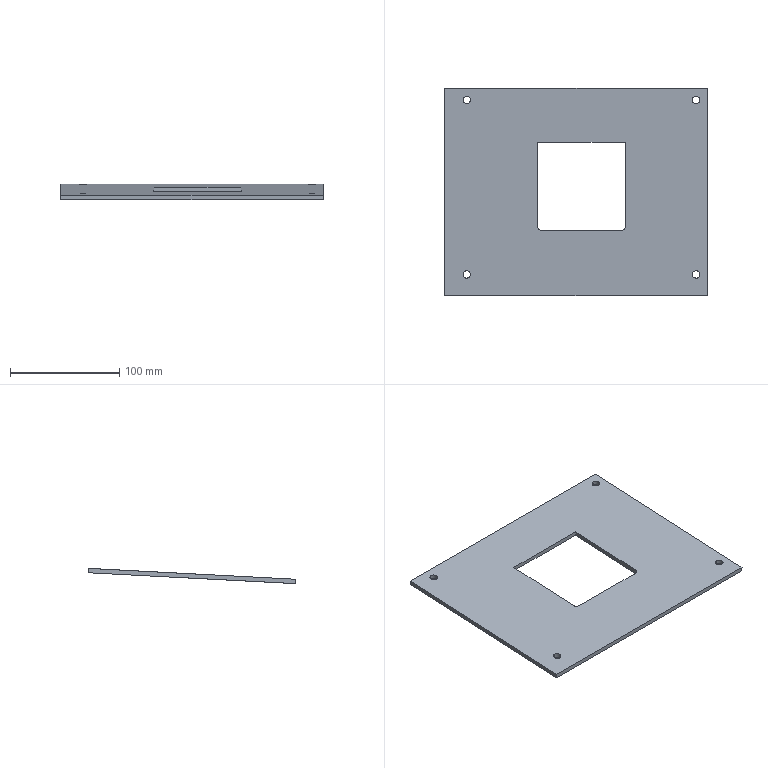Component | SolidWorks | YC1-315HangingBoxOverall-1_YC1-315SupportFrameT()-1_YC1-160OperationStationBaffleT-1 | 1 solid | 20 faces | box 240 x 189.95 x 13.94 mm | volume 155860 mm3 | cylinder 10 | plane 10 | commonest cylinder face diameters 7 x8 8 x2 | material Plain Carbon Steel
STEP:
#1=COLOUR_RGB('',0.7922,0.8196,0.9333);
#2=FILL_AREA_STYLE_COLOUR('',#1);
#3=FILL_AREA_STYLE('',(#2));
#4=SURFACE_STYLE_FILL_AREA(#3);
#5=SURFACE_SIDE_STYLE('',(#4));
#6=SURFACE_STYLE_USAGE(.BOTH.,#5);
#7=PRESENTATION_STYLE_ASSIGNMENT((#6));
#8=CARTESIAN_POINT('',(33.071,65.604,2.308));
#9=VERTEX_POINT('',#8);
#10=CARTESIAN_POINT('',(33.071,65.328,2.294));
#11=VERTEX_POINT('',#10);
#12=CARTESIAN_POINT('',(33.071,65.466,2.301));
#13=DIRECTION('',(-0.,-0.05234,0.9986));
#14=DIRECTION('',(0.,-0.9986,-0.05234));
#15=AXIS2_PLACEMENT_3D('',#12,#13,#14);
#16=CIRCLE('',#15,0.1378);
#17=EDGE_CURVE('',#9,#11,#16,.T.);
#18=ORIENTED_EDGE('',*,*,#17,.F.);
#19=CARTESIAN_POINT('',(33.071,65.595,2.465));
#20=VERTEX_POINT('',#19);
#21=CARTESIAN_POINT('',(33.071,65.604,2.308));
#22=DIRECTION('',(-0.,-0.05234,0.9986));
#23=VECTOR('',#22,39.37);
#24=LINE('',#21,#23);
#25=EDGE_CURVE('',#9,#20,#24,.T.);
#26=ORIENTED_EDGE('',*,*,#25,.T.);
#27=CARTESIAN_POINT('',(33.071,65.32,2.451));
#28=VERTEX_POINT('',#27);
#29=CARTESIAN_POINT('',(33.071,65.458,2.458));
#30=DIRECTION('',(-0.,-0.05234,0.9986));
#31=DIRECTION('',(0.,-0.9986,-0.05234));
#32=AXIS2_PLACEMENT_3D('',#29,#30,#31);
#33=CIRCLE('',#32,0.1378);
#34=EDGE_CURVE('',#20,#28,#33,.T.);
#35=ORIENTED_EDGE('',*,*,#34,.T.);
#36=CARTESIAN_POINT('',(33.071,65.328,2.294));
#37=DIRECTION('',(-0.,-0.05234,0.9986));
#38=VECTOR('',#37,39.37);
#39=LINE('',#36,#38);
#40=EDGE_CURVE('',#11,#28,#39,.T.);
#41=ORIENTED_EDGE('',*,*,#40,.F.);
#42=EDGE_LOOP('',(#18,#26,#35,#41));
#43=FACE_OUTER_BOUND('',#42,.T.);
#44=CARTESIAN_POINT('',(33.071,65.466,2.301));
#45=DIRECTION('',(-0.,-0.05234,0.9986));
#46=DIRECTION('',(0.,-0.9986,-0.05234));
#47=AXIS2_PLACEMENT_3D('',#44,#45,#46);
#48=CYLINDRICAL_SURFACE('',#47,0.1378);
#49=ADVANCED_FACE('',(#43),#48,.F.);
#50=CARTESIAN_POINT('',(41.339,65.604,2.308));
#51=VERTEX_POINT('',#50);
#52=CARTESIAN_POINT('',(41.339,65.328,2.294));
#53=VERTEX_POINT('',#52);
#54=CARTESIAN_POINT('',(41.339,65.466,2.301));
#55=DIRECTION('',(-0.,-0.05234,0.9986));
#56=DIRECTION('',(0.,-0.9986,-0.05234));
#57=AXIS2_PLACEMENT_3D('',#54,#55,#56);
#58=CIRCLE('',#57,0.1378);
#59=EDGE_CURVE('',#51,#53,#58,.T.);
#60=ORIENTED_EDGE('',*,*,#59,.F.);
#61=CARTESIAN_POINT('',(41.339,65.595,2.465));
#62=VERTEX_POINT('',#61);
#63=CARTESIAN_POINT('',(41.339,65.604,2.308));
#64=DIRECTION('',(-0.,-0.05234,0.9986));
#65=VECTOR('',#64,39.37);
#66=LINE('',#63,#65);
#67=EDGE_CURVE('',#51,#62,#66,.T.);
#68=ORIENTED_EDGE('',*,*,#67,.T.);
#69=CARTESIAN_POINT('',(41.339,65.32,2.451));
#70=VERTEX_POINT('',#69);
#71=CARTESIAN_POINT('',(41.339,65.458,2.458));
#72=DIRECTION('',(-0.,-0.05234,0.9986));
#73=DIRECTION('',(0.,-0.9986,-0.05234));
#74=AXIS2_PLACEMENT_3D('',#71,#72,#73);
#75=CIRCLE('',#74,0.1378);
#76=EDGE_CURVE('',#62,#70,#75,.T.);
#77=ORIENTED_EDGE('',*,*,#76,.T.);
#78=CARTESIAN_POINT('',(41.339,65.328,2.294));
#79=DIRECTION('',(-0.,-0.05234,0.9986));
#80=VECTOR('',#79,39.37);
#81=LINE('',#78,#80);
#82=EDGE_CURVE('',#53,#70,#81,.T.);
#83=ORIENTED_EDGE('',*,*,#82,.F.);
#84=EDGE_LOOP('',(#60,#68,#77,#83));
#85=FACE_OUTER_BOUND('',#84,.T.);
#86=CARTESIAN_POINT('',(41.339,65.466,2.301));
#87=DIRECTION('',(-0.,-0.05234,0.9986));
#88=DIRECTION('',(0.,-0.9986,-0.05234));
#89=AXIS2_PLACEMENT_3D('',#86,#87,#88);
#90=CYLINDRICAL_SURFACE('',#89,0.1378);
#91=ADVANCED_FACE('',(#85),#90,.F.);
#92=CARTESIAN_POINT('',(41.339,59.313,1.978));
#93=VERTEX_POINT('',#92);
#94=CARTESIAN_POINT('',(41.339,59.038,1.964));
#95=VERTEX_POINT('',#94);
#96=CARTESIAN_POINT('',(41.339,59.175,1.971));
#97=DIRECTION('',(-0.,-0.05234,0.9986));
#98=DIRECTION('',(0.,-0.9986,-0.05234));
#99=AXIS2_PLACEMENT_3D('',#96,#97,#98);
#100=CIRCLE('',#99,0.1378);
#101=EDGE_CURVE('',#93,#95,#100,.T.);
#102=ORIENTED_EDGE('',*,*,#101,.F.);
#103=CARTESIAN_POINT('',(41.339,59.305,2.136));
#104=VERTEX_POINT('',#103);
#105=CARTESIAN_POINT('',(41.339,59.313,1.978));
#106=DIRECTION('',(-0.,-0.05234,0.9986));
#107=VECTOR('',#106,39.37);
#108=LINE('',#105,#107);
#109=EDGE_CURVE('',#93,#104,#108,.T.);
#110=ORIENTED_EDGE('',*,*,#109,.T.);
#111=CARTESIAN_POINT('',(41.339,59.03,2.121));
#112=VERTEX_POINT('',#111);
#113=CARTESIAN_POINT('',(41.339,59.167,2.128));
#114=DIRECTION('',(-0.,-0.05234,0.9986));
#115=DIRECTION('',(0.,-0.9986,-0.05234));
#116=AXIS2_PLACEMENT_3D('',#113,#114,#115);
#117=CIRCLE('',#116,0.1378);
#118=EDGE_CURVE('',#104,#112,#117,.T.);
#119=ORIENTED_EDGE('',*,*,#118,.T.);
#120=CARTESIAN_POINT('',(41.339,59.038,1.964));
#121=DIRECTION('',(-0.,-0.05234,0.9986));
#122=VECTOR('',#121,39.37);
#123=LINE('',#120,#122);
#124=EDGE_CURVE('',#95,#112,#123,.T.);
#125=ORIENTED_EDGE('',*,*,#124,.F.);
#126=EDGE_LOOP('',(#102,#110,#119,#125));
#127=FACE_OUTER_BOUND('',#126,.T.);
#128=CARTESIAN_POINT('',(41.339,59.175,1.971));
#129=DIRECTION('',(-0.,-0.05234,0.9986));
#130=DIRECTION('',(0.,-0.9986,-0.05234));
#131=AXIS2_PLACEMENT_3D('',#128,#129,#130);
#132=CYLINDRICAL_SURFACE('',#131,0.1378);
#133=ADVANCED_FACE('',(#127),#132,.F.);
#134=CARTESIAN_POINT('',(33.071,59.313,1.978));
#135=VERTEX_POINT('',#134);
#136=CARTESIAN_POINT('',(33.071,59.038,1.964));
#137=VERTEX_POINT('',#136);
#138=CARTESIAN_POINT('',(33.071,59.175,1.971));
#139=DIRECTION('',(-0.,-0.05234,0.9986));
#140=DIRECTION('',(0.,-0.9986,-0.05234));
#141=AXIS2_PLACEMENT_3D('',#138,#139,#140);
#142=CIRCLE('',#141,0.1378);
#143=EDGE_CURVE('',#135,#137,#142,.T.);
#144=ORIENTED_EDGE('',*,*,#143,.F.);
#145=CARTESIAN_POINT('',(33.071,59.305,2.136));
#146=VERTEX_POINT('',#145);
#147=CARTESIAN_POINT('',(33.071,59.313,1.978));
#148=DIRECTION('',(-0.,-0.05234,0.9986));
#149=VECTOR('',#148,39.37);
#150=LINE('',#147,#149);
#151=EDGE_CURVE('',#135,#146,#150,.T.);
#152=ORIENTED_EDGE('',*,*,#151,.T.);
#153=CARTESIAN_POINT('',(33.071,59.03,2.121));
#154=VERTEX_POINT('',#153);
#155=CARTESIAN_POINT('',(33.071,59.167,2.128));
#156=DIRECTION('',(-0.,-0.05234,0.9986));
#157=DIRECTION('',(0.,-0.9986,-0.05234));
#158=AXIS2_PLACEMENT_3D('',#155,#156,#157);
#159=CIRCLE('',#158,0.1378);
#160=EDGE_CURVE('',#146,#154,#159,.T.);
#161=ORIENTED_EDGE('',*,*,#160,.T.);
#162=CARTESIAN_POINT('',(33.071,59.038,1.964));
#163=DIRECTION('',(-0.,-0.05234,0.9986));
#164=VECTOR('',#163,39.37);
#165=LINE('',#162,#164);
#166=EDGE_CURVE('',#137,#154,#165,.T.);
#167=ORIENTED_EDGE('',*,*,#166,.F.);
#168=EDGE_LOOP('',(#144,#152,#161,#167));
#169=FACE_OUTER_BOUND('',#168,.T.);
#170=CARTESIAN_POINT('',(33.071,59.175,1.971));
#171=DIRECTION('',(-0.,-0.05234,0.9986));
#172=DIRECTION('',(0.,-0.9986,-0.05234));
#173=AXIS2_PLACEMENT_3D('',#170,#171,#172);
#174=CYLINDRICAL_SURFACE('',#173,0.1378);
#175=ADVANCED_FACE('',(#169),#174,.F.);
#176=CARTESIAN_POINT('',(35.63,63.928,2.378));
#177=VERTEX_POINT('',#176);
#178=CARTESIAN_POINT('',(35.63,60.897,2.219));
#179=VERTEX_POINT('',#178);
#180=CARTESIAN_POINT('',(35.63,65.871,2.48));
#181=DIRECTION('',(0.,-0.9986,-0.05234));
#182=VECTOR('',#181,39.37);
#183=LINE('',#180,#182);
#184=EDGE_CURVE('',#177,#179,#183,.T.);
#185=ORIENTED_EDGE('',*,*,#184,.F.);
#186=CARTESIAN_POINT('',(38.78,63.928,2.378));
#187=VERTEX_POINT('',#186);
#188=CARTESIAN_POINT('',(32.283,63.928,2.378));
#189=DIRECTION('',(1.,0.,0.));
#190=VECTOR('',#189,39.37);
#191=LINE('',#188,#190);
#192=EDGE_CURVE('',#177,#187,#191,.T.);
#193=ORIENTED_EDGE('',*,*,#192,.T.);
#194=CARTESIAN_POINT('',(38.78,60.897,2.219));
#195=VERTEX_POINT('',#194);
#196=CARTESIAN_POINT('',(38.78,65.871,2.48));
#197=DIRECTION('',(-0.,0.9986,0.05234));
#198=VECTOR('',#197,39.37);
#199=LINE('',#196,#198);
#200=EDGE_CURVE('',#195,#187,#199,.T.);
#201=ORIENTED_EDGE('',*,*,#200,.F.);
#202=CARTESIAN_POINT('',(38.622,60.74,2.211));
#203=VERTEX_POINT('',#202);
#204=CARTESIAN_POINT('',(38.622,60.897,2.219));
#205=DIRECTION('',(-0.,-0.05234,0.9986));
#206=DIRECTION('',(0.,-0.9986,-0.05234));
#207=AXIS2_PLACEMENT_3D('',#204,#205,#206);
#208=CIRCLE('',#207,0.1575);
#209=EDGE_CURVE('',#203,#195,#208,.T.);
#210=ORIENTED_EDGE('',*,*,#209,.F.);
#211=CARTESIAN_POINT('',(35.787,60.74,2.211));
#212=VERTEX_POINT('',#211);
#213=CARTESIAN_POINT('',(32.283,60.74,2.211));
#214=DIRECTION('',(1.,0.,0.));
#215=VECTOR('',#214,39.37);
#216=LINE('',#213,#215);
#217=EDGE_CURVE('',#212,#203,#216,.T.);
#218=ORIENTED_EDGE('',*,*,#217,.F.);
#219=CARTESIAN_POINT('',(35.787,60.897,2.219));
#220=DIRECTION('',(-0.,-0.05234,0.9986));
#221=DIRECTION('',(0.,-0.9986,-0.05234));
#222=AXIS2_PLACEMENT_3D('',#219,#220,#221);
#223=CIRCLE('',#222,0.1575);
#224=EDGE_CURVE('',#179,#212,#223,.T.);
#225=ORIENTED_EDGE('',*,*,#224,.F.);
#226=EDGE_LOOP('',(#185,#193,#201,#210,#218,#225));
#227=FACE_BOUND('',#226,.T.);
#228=CARTESIAN_POINT('',(41.732,58.4,2.088));
#229=VERTEX_POINT('',#228);
#230=CARTESIAN_POINT('',(32.283,58.4,2.088));
#231=VERTEX_POINT('',#230);
#232=CARTESIAN_POINT('',(32.283,58.4,2.088));
#233=DIRECTION('',(-1.,-0.,-0.));
#234=VECTOR('',#233,39.37);
#235=LINE('',#232,#234);
#236=EDGE_CURVE('',#229,#231,#235,.T.);
#237=ORIENTED_EDGE('',*,*,#236,.F.);
#238=CARTESIAN_POINT('',(41.732,65.871,2.48));
#239=VERTEX_POINT('',#238);
#240=CARTESIAN_POINT('',(41.732,65.871,2.48));
#241=DIRECTION('',(0.,-0.9986,-0.05234));
#242=VECTOR('',#241,39.37);
#243=LINE('',#240,#242);
#244=EDGE_CURVE('',#239,#229,#243,.T.);
#245=ORIENTED_EDGE('',*,*,#244,.F.);
#246=CARTESIAN_POINT('',(32.283,65.871,2.48));
#247=VERTEX_POINT('',#246);
#248=CARTESIAN_POINT('',(32.283,65.871,2.48));
#249=DIRECTION('',(1.,0.,0.));
#250=VECTOR('',#249,39.37);
#251=LINE('',#248,#250);
#252=EDGE_CURVE('',#247,#239,#251,.T.);
#253=ORIENTED_EDGE('',*,*,#252,.F.);
#254=CARTESIAN_POINT('',(32.283,65.871,2.48));
#255=DIRECTION('',(-0.,0.9986,0.05234));
#256=VECTOR('',#255,39.37);
#257=LINE('',#254,#256);
#258=EDGE_CURVE('',#231,#247,#257,.T.);
#259=ORIENTED_EDGE('',*,*,#258,.F.);
#260=EDGE_LOOP('',(#237,#245,#253,#259));
#261=FACE_OUTER_BOUND('',#260,.T.);
#262=CARTESIAN_POINT('',(33.071,65.458,2.458));
#263=DIRECTION('',(-0.,-0.05234,0.9986));
#264=DIRECTION('',(0.,-0.9986,-0.05234));
#265=AXIS2_PLACEMENT_3D('',#262,#263,#264);
#266=CIRCLE('',#265,0.1378);
#267=EDGE_CURVE('',#28,#20,#266,.T.);
#268=ORIENTED_EDGE('',*,*,#267,.F.);
#269=ORIENTED_EDGE('',*,*,#34,.F.);
#270=EDGE_LOOP('',(#268,#269));
#271=FACE_BOUND('',#270,.T.);
#272=CARTESIAN_POINT('',(41.339,65.458,2.458));
#273=DIRECTION('',(-0.,-0.05234,0.9986));
#274=DIRECTION('',(0.,-0.9986,-0.05234));
#275=AXIS2_PLACEMENT_3D('',#272,#273,#274);
#276=CIRCLE('',#275,0.1378);
#277=EDGE_CURVE('',#70,#62,#276,.T.);
#278=ORIENTED_EDGE('',*,*,#277,.F.);
#279=ORIENTED_EDGE('',*,*,#76,.F.);
#280=EDGE_LOOP('',(#278,#279));
#281=FACE_BOUND('',#280,.T.);
#282=CARTESIAN_POINT('',(41.339,59.167,2.128));
#283=DIRECTION('',(-0.,-0.05234,0.9986));
#284=DIRECTION('',(0.,-0.9986,-0.05234));
#285=AXIS2_PLACEMENT_3D('',#282,#283,#284);
#286=CIRCLE('',#285,0.1378);
#287=EDGE_CURVE('',#112,#104,#286,.T.);
#288=ORIENTED_EDGE('',*,*,#287,.F.);
#289=ORIENTED_EDGE('',*,*,#118,.F.);
#290=EDGE_LOOP('',(#288,#289));
#291=FACE_BOUND('',#290,.T.);
#292=CARTESIAN_POINT('',(33.071,59.167,2.128));
#293=DIRECTION('',(-0.,-0.05234,0.9986));
#294=DIRECTION('',(0.,-0.9986,-0.05234));
#295=AXIS2_PLACEMENT_3D('',#292,#293,#294);
#296=CIRCLE('',#295,0.1378);
#297=EDGE_CURVE('',#154,#146,#296,.T.);
#298=ORIENTED_EDGE('',*,*,#297,.F.);
#299=ORIENTED_EDGE('',*,*,#160,.F.);
#300=EDGE_LOOP('',(#298,#299));
#301=FACE_BOUND('',#300,.T.);
#302=CARTESIAN_POINT('',(32.283,65.871,2.48));
#303=DIRECTION('',(0.,0.05234,-0.9986));
#304=DIRECTION('',(-0.,0.9986,0.05234));
#305=AXIS2_PLACEMENT_3D('',#302,#303,#304);
#306=PLANE('',#305);
#307=ADVANCED_FACE('',(#227,#261,#271,#281,#291,#301),#306,.F.);
#308=ORIENTED_EDGE('',*,*,#184,.T.);
#309=CARTESIAN_POINT('',(35.63,60.905,2.062));
#310=VERTEX_POINT('',#309);
#311=CARTESIAN_POINT('',(35.63,60.897,2.219));
#312=DIRECTION('',(0.,0.05234,-0.9986));
#313=VECTOR('',#312,39.37);
#314=LINE('',#311,#313);
#315=EDGE_CURVE('',#179,#310,#314,.T.);
#316=ORIENTED_EDGE('',*,*,#315,.T.);
#317=CARTESIAN_POINT('',(35.63,63.937,2.221));
#318=VERTEX_POINT('',#317);
#319=CARTESIAN_POINT('',(35.63,63.893,2.218));
#320=DIRECTION('',(-0.,0.9986,0.05234));
#321=VECTOR('',#320,39.37);
#322=LINE('',#319,#321);
#323=EDGE_CURVE('',#310,#318,#322,.T.);
#324=ORIENTED_EDGE('',*,*,#323,.T.);
#325=CARTESIAN_POINT('',(35.63,63.998,1.041));
#326=DIRECTION('',(-0.,-0.05234,0.9986));
#327=VECTOR('',#326,39.37);
#328=LINE('',#325,#327);
#329=EDGE_CURVE('',#318,#177,#328,.T.);
#330=ORIENTED_EDGE('',*,*,#329,.T.);
#331=EDGE_LOOP('',(#308,#316,#324,#330));
#332=FACE_OUTER_BOUND('',#331,.T.);
#333=CARTESIAN_POINT('',(35.63,63.885,2.376));
#334=DIRECTION('',(1.,0.,0.));
#335=DIRECTION('',(-0.,0.9986,0.05234));
#336=AXIS2_PLACEMENT_3D('',#333,#334,#335);
#337=PLANE('',#336);
#338=ADVANCED_FACE('',(#332),#337,.T.);
#339=ORIENTED_EDGE('',*,*,#200,.T.);
#340=CARTESIAN_POINT('',(38.78,63.937,2.221));
#341=VERTEX_POINT('',#340);
#342=CARTESIAN_POINT('',(38.78,63.998,1.041));
#343=DIRECTION('',(-0.,-0.05234,0.9986));
#344=VECTOR('',#343,39.37);
#345=LINE('',#342,#344);
#346=EDGE_CURVE('',#341,#187,#345,.T.);
#347=ORIENTED_EDGE('',*,*,#346,.F.);
#348=CARTESIAN_POINT('',(38.78,60.905,2.062));
#349=VERTEX_POINT('',#348);
#350=CARTESIAN_POINT('',(38.78,63.893,2.218));
#351=DIRECTION('',(0.,-0.9986,-0.05234));
#352=VECTOR('',#351,39.37);
#353=LINE('',#350,#352);
#354=EDGE_CURVE('',#341,#349,#353,.T.);
#355=ORIENTED_EDGE('',*,*,#354,.T.);
#356=CARTESIAN_POINT('',(38.78,60.897,2.219));
#357=DIRECTION('',(-0.,-0.05234,0.9986));
#358=VECTOR('',#357,39.37);
#359=LINE('',#356,#358);
#360=EDGE_CURVE('',#349,#195,#359,.T.);
#361=ORIENTED_EDGE('',*,*,#360,.T.);
#362=EDGE_LOOP('',(#339,#347,#355,#361));
#363=FACE_OUTER_BOUND('',#362,.T.);
#364=CARTESIAN_POINT('',(38.78,63.885,2.376));
#365=DIRECTION('',(-1.,-0.,-0.));
#366=DIRECTION('',(-0.,-0.05234,0.9986));
#367=AXIS2_PLACEMENT_3D('',#364,#365,#366);
#368=PLANE('',#367);
#369=ADVANCED_FACE('',(#363),#368,.T.);
#370=ORIENTED_EDGE('',*,*,#360,.F.);
#371=CARTESIAN_POINT('',(38.622,60.748,2.053));
#372=VERTEX_POINT('',#371);
#373=CARTESIAN_POINT('',(38.622,60.905,2.062));
#374=DIRECTION('',(-0.,-0.05234,0.9986));
#375=DIRECTION('',(0.,-0.9986,-0.05234));
#376=AXIS2_PLACEMENT_3D('',#373,#374,#375);
#377=CIRCLE('',#376,0.1575);
#378=EDGE_CURVE('',#372,#349,#377,.T.);
#379=ORIENTED_EDGE('',*,*,#378,.F.);
#380=CARTESIAN_POINT('',(38.622,60.74,2.211));
#381=DIRECTION('',(0.,0.05234,-0.9986));
#382=VECTOR('',#381,39.37);
#383=LINE('',#380,#382);
#384=EDGE_CURVE('',#203,#372,#383,.T.);
#385=ORIENTED_EDGE('',*,*,#384,.F.);
#386=ORIENTED_EDGE('',*,*,#209,.T.);
#387=EDGE_LOOP('',(#370,#379,#385,#386));
#388=FACE_OUTER_BOUND('',#387,.T.);
#389=CARTESIAN_POINT('',(38.622,60.897,2.219));
#390=DIRECTION('',(-0.,-0.05234,0.9986));
#391=DIRECTION('',(0.,-0.9986,-0.05234));
#392=AXIS2_PLACEMENT_3D('',#389,#390,#391);
#393=CYLINDRICAL_SURFACE('',#392,0.1575);
#394=ADVANCED_FACE('',(#388),#393,.F.);
#395=CARTESIAN_POINT('',(35.787,60.748,2.053));
#396=VERTEX_POINT('',#395);
#397=CARTESIAN_POINT('',(35.63,60.748,2.053));
#398=DIRECTION('',(-1.,-0.,-0.));
#399=VECTOR('',#398,39.37);
#400=LINE('',#397,#399);
#401=EDGE_CURVE('',#372,#396,#400,.T.);
#402=ORIENTED_EDGE('',*,*,#401,.T.);
#403=CARTESIAN_POINT('',(35.787,60.74,2.211));
#404=DIRECTION('',(-0.,-0.05234,0.9986));
#405=VECTOR('',#404,39.37);
#406=LINE('',#403,#405);
#407=EDGE_CURVE('',#396,#212,#406,.T.);
#408=ORIENTED_EDGE('',*,*,#407,.T.);
#409=ORIENTED_EDGE('',*,*,#217,.T.);
#410=ORIENTED_EDGE('',*,*,#384,.T.);
#411=EDGE_LOOP('',(#402,#408,#409,#410));
#412=FACE_OUTER_BOUND('',#411,.T.);
#413=CARTESIAN_POINT('',(35.63,60.74,2.211));
#414=DIRECTION('',(-0.,0.9986,0.05234));
#415=DIRECTION('',(-0.,-0.05234,0.9986));
#416=AXIS2_PLACEMENT_3D('',#413,#414,#415);
#417=PLANE('',#416);
#418=ADVANCED_FACE('',(#412),#417,.T.);
#419=ORIENTED_EDGE('',*,*,#407,.F.);
#420=CARTESIAN_POINT('',(35.787,60.905,2.062));
#421=DIRECTION('',(-0.,-0.05234,0.9986));
#422=DIRECTION('',(0.,-0.9986,-0.05234));
#423=AXIS2_PLACEMENT_3D('',#420,#421,#422);
#424=CIRCLE('',#423,0.1575);
#425=EDGE_CURVE('',#310,#396,#424,.T.);
#426=ORIENTED_EDGE('',*,*,#425,.F.);
#427=ORIENTED_EDGE('',*,*,#315,.F.);
#428=ORIENTED_EDGE('',*,*,#224,.T.);
#429=EDGE_LOOP('',(#419,#426,#427,#428));
#430=FACE_OUTER_BOUND('',#429,.T.);
#431=CARTESIAN_POINT('',(35.787,60.897,2.219));
#432=DIRECTION('',(-0.,-0.05234,0.9986));
#433=DIRECTION('',(0.,-0.9986,-0.05234));
#434=AXIS2_PLACEMENT_3D('',#431,#432,#433);
#435=CYLINDRICAL_SURFACE('',#434,0.1575);
#436=ADVANCED_FACE('',(#430),#435,.F.);
#437=CARTESIAN_POINT('',(32.283,58.409,1.931));
#438=VERTEX_POINT('',#437);
#439=CARTESIAN_POINT('',(32.283,58.4,2.088));
#440=DIRECTION('',(0.,0.05234,-0.9986));
#441=VECTOR('',#440,39.37);
#442=LINE('',#439,#441);
#443=EDGE_CURVE('',#231,#438,#442,.T.);
#444=ORIENTED_EDGE('',*,*,#443,.F.);
#445=ORIENTED_EDGE('',*,*,#258,.T.);
#446=CARTESIAN_POINT('',(32.283,65.879,2.322));
#447=VERTEX_POINT('',#446);
#448=CARTESIAN_POINT('',(32.283,65.871,2.48));
#449=DIRECTION('',(-0.,-0.05234,0.9986));
#450=VECTOR('',#449,39.37);
#451=LINE('',#448,#450);
#452=EDGE_CURVE('',#447,#247,#451,.T.);
#453=ORIENTED_EDGE('',*,*,#452,.F.);
#454=CARTESIAN_POINT('',(32.283,58.409,1.931));
#455=DIRECTION('',(-0.,0.9986,0.05234));
#456=VECTOR('',#455,39.37);
#457=LINE('',#454,#456);
#458=EDGE_CURVE('',#438,#447,#457,.T.);
#459=ORIENTED_EDGE('',*,*,#458,.F.);
#460=EDGE_LOOP('',(#444,#445,#453,#459));
#461=FACE_OUTER_BOUND('',#460,.T.);
#462=CARTESIAN_POINT('',(32.283,58.4,2.088));
#463=DIRECTION('',(1.,0.,0.));
#464=DIRECTION('',(0.,0.05234,-0.9986));
#465=AXIS2_PLACEMENT_3D('',#462,#463,#464);
#466=PLANE('',#465);
#467=ADVANCED_FACE('',(#461),#466,.F.);
#468=CARTESIAN_POINT('',(41.732,58.409,1.931));
#469=VERTEX_POINT('',#468);
#470=CARTESIAN_POINT('',(41.732,58.4,2.088));
#471=DIRECTION('',(0.,0.05234,-0.9986));
#472=VECTOR('',#471,39.37);
#473=LINE('',#470,#472);
#474=EDGE_CURVE('',#229,#469,#473,.T.);
#475=ORIENTED_EDGE('',*,*,#474,.F.);
#476=ORIENTED_EDGE('',*,*,#236,.T.);
#477=ORIENTED_EDGE('',*,*,#443,.T.);
#478=CARTESIAN_POINT('',(32.283,58.409,1.931));
#479=DIRECTION('',(-1.,-0.,-0.));
#480=VECTOR('',#479,39.37);
#481=LINE('',#478,#480);
#482=EDGE_CURVE('',#469,#438,#481,.T.);
#483=ORIENTED_EDGE('',*,*,#482,.F.);
#484=EDGE_LOOP('',(#475,#476,#477,#483));
#485=FACE_OUTER_BOUND('',#484,.T.);
#486=CARTESIAN_POINT('',(32.283,58.4,2.088));
#487=DIRECTION('',(-0.,0.9986,0.05234));
#488=DIRECTION('',(-0.,-0.05234,0.9986));
#489=AXIS2_PLACEMENT_3D('',#486,#487,#488);
#490=PLANE('',#489);
#491=ADVANCED_FACE('',(#485),#490,.F.);
#492=CARTESIAN_POINT('',(41.732,65.879,2.322));
#493=VERTEX_POINT('',#492);
#494=CARTESIAN_POINT('',(41.732,65.871,2.48));
#495=DIRECTION('',(0.,0.05234,-0.9986));
#496=VECTOR('',#495,39.37);
#497=LINE('',#494,#496);
#498=EDGE_CURVE('',#239,#493,#497,.T.);
#499=ORIENTED_EDGE('',*,*,#498,.F.);
#500=ORIENTED_EDGE('',*,*,#244,.T.);
#501=ORIENTED_EDGE('',*,*,#474,.T.);
#502=CARTESIAN_POINT('',(41.732,58.409,1.931));
#503=DIRECTION('',(0.,-0.9986,-0.05234));
#504=VECTOR('',#503,39.37);
#505=LINE('',#502,#504);
#506=EDGE_CURVE('',#493,#469,#505,.T.);
#507=ORIENTED_EDGE('',*,*,#506,.F.);
#508=EDGE_LOOP('',(#499,#500,#501,#507));
#509=FACE_OUTER_BOUND('',#508,.T.);
#510=CARTESIAN_POINT('',(41.732,58.4,2.088));
#511=DIRECTION('',(-1.,-0.,-0.));
#512=DIRECTION('',(-0.,-0.05234,0.9986));
#513=AXIS2_PLACEMENT_3D('',#510,#511,#512);
#514=PLANE('',#513);
#515=ADVANCED_FACE('',(#509),#514,.F.);
#516=ORIENTED_EDGE('',*,*,#452,.T.);
#517=ORIENTED_EDGE('',*,*,#252,.T.);
#518=ORIENTED_EDGE('',*,*,#498,.T.);
#519=CARTESIAN_POINT('',(32.283,65.879,2.322));
#520=DIRECTION('',(1.,0.,0.));
#521=VECTOR('',#520,39.37);
#522=LINE('',#519,#521);
#523=EDGE_CURVE('',#447,#493,#522,.T.);
#524=ORIENTED_EDGE('',*,*,#523,.F.);
#525=EDGE_LOOP('',(#516,#517,#518,#524));
#526=FACE_OUTER_BOUND('',#525,.T.);
#527=CARTESIAN_POINT('',(32.283,65.871,2.48));
#528=DIRECTION('',(0.,-0.9986,-0.05234));
#529=DIRECTION('',(0.,0.05234,-0.9986));
#530=AXIS2_PLACEMENT_3D('',#527,#528,#529);
#531=PLANE('',#530);
#532=ADVANCED_FACE('',(#526),#531,.F.);
#533=ORIENTED_EDGE('',*,*,#25,.F.);
#534=CARTESIAN_POINT('',(33.071,65.466,2.301));
#535=DIRECTION('',(-0.,-0.05234,0.9986));
#536=DIRECTION('',(0.,-0.9986,-0.05234));
#537=AXIS2_PLACEMENT_3D('',#534,#535,#536);
#538=CIRCLE('',#537,0.1378);
#539=EDGE_CURVE('',#11,#9,#538,.T.);
#540=ORIENTED_EDGE('',*,*,#539,.F.);
#541=ORIENTED_EDGE('',*,*,#40,.T.);
#542=ORIENTED_EDGE('',*,*,#267,.T.);
#543=EDGE_LOOP('',(#533,#540,#541,#542));
#544=FACE_OUTER_BOUND('',#543,.T.);
#545=CARTESIAN_POINT('',(33.071,65.466,2.301));
#546=DIRECTION('',(-0.,-0.05234,0.9986));
#547=DIRECTION('',(0.,-0.9986,-0.05234));
#548=AXIS2_PLACEMENT_3D('',#545,#546,#547);
#549=CYLINDRICAL_SURFACE('',#548,0.1378);
#550=ADVANCED_FACE('',(#544),#549,.F.);
#551=ORIENTED_EDGE('',*,*,#67,.F.);
#552=CARTESIAN_POINT('',(41.339,65.466,2.301));
#553=DIRECTION('',(-0.,-0.05234,0.9986));
#554=DIRECTION('',(0.,-0.9986,-0.05234));
#555=AXIS2_PLACEMENT_3D('',#552,#553,#554);
#556=CIRCLE('',#555,0.1378);
#557=EDGE_CURVE('',#53,#51,#556,.T.);
#558=ORIENTED_EDGE('',*,*,#557,.F.);
#559=ORIENTED_EDGE('',*,*,#82,.T.);
#560=ORIENTED_EDGE('',*,*,#277,.T.);
#561=EDGE_LOOP('',(#551,#558,#559,#560));
#562=FACE_OUTER_BOUND('',#561,.T.);
#563=CARTESIAN_POINT('',(41.339,65.466,2.301));
#564=DIRECTION('',(-0.,-0.05234,0.9986));
#565=DIRECTION('',(0.,-0.9986,-0.05234));
#566=AXIS2_PLACEMENT_3D('',#563,#564,#565);
#567=CYLINDRICAL_SURFACE('',#566,0.1378);
#568=ADVANCED_FACE('',(#562),#567,.F.);
#569=ORIENTED_EDGE('',*,*,#109,.F.);
#570=CARTESIAN_POINT('',(41.339,59.175,1.971));
#571=DIRECTION('',(-0.,-0.05234,0.9986));
#572=DIRECTION('',(0.,-0.9986,-0.05234));
#573=AXIS2_PLACEMENT_3D('',#570,#571,#572);
#574=CIRCLE('',#573,0.1378);
#575=EDGE_CURVE('',#95,#93,#574,.T.);
#576=ORIENTED_EDGE('',*,*,#575,.F.);
#577=ORIENTED_EDGE('',*,*,#124,.T.);
#578=ORIENTED_EDGE('',*,*,#287,.T.);
#579=EDGE_LOOP('',(#569,#576,#577,#578));
#580=FACE_OUTER_BOUND('',#579,.T.);
#581=CARTESIAN_POINT('',(41.339,59.175,1.971));
#582=DIRECTION('',(-0.,-0.05234,0.9986));
#583=DIRECTION('',(0.,-0.9986,-0.05234));
#584=AXIS2_PLACEMENT_3D('',#581,#582,#583);
#585=CYLINDRICAL_SURFACE('',#584,0.1378);
#586=ADVANCED_FACE('',(#580),#585,.F.);
#587=ORIENTED_EDGE('',*,*,#151,.F.);
#588=CARTESIAN_POINT('',(33.071,59.175,1.971));
#589=DIRECTION('',(-0.,-0.05234,0.9986));
#590=DIRECTION('',(0.,-0.9986,-0.05234));
#591=AXIS2_PLACEMENT_3D('',#588,#589,#590);
#592=CIRCLE('',#591,0.1378);
#593=EDGE_CURVE('',#137,#135,#592,.T.);
#594=ORIENTED_EDGE('',*,*,#593,.F.);
#595=ORIENTED_EDGE('',*,*,#166,.T.);
#596=ORIENTED_EDGE('',*,*,#297,.T.);
#597=EDGE_LOOP('',(#587,#594,#595,#596));
#598=FACE_OUTER_BOUND('',#597,.T.);
#599=CARTESIAN_POINT('',(33.071,59.175,1.971));
#600=DIRECTION('',(-0.,-0.05234,0.9986));
#601=DIRECTION('',(0.,-0.9986,-0.05234));
#602=AXIS2_PLACEMENT_3D('',#599,#600,#601);
#603=CYLINDRICAL_SURFACE('',#602,0.1378);
#604=ADVANCED_FACE('',(#598),#603,.F.);
#605=CARTESIAN_POINT('',(32.283,63.937,2.221));
#606=DIRECTION('',(1.,0.,0.));
#607=VECTOR('',#606,39.37);
#608=LINE('',#605,#607);
#609=EDGE_CURVE('',#318,#341,#608,.T.);
#610=ORIENTED_EDGE('',*,*,#609,.F.);
#611=ORIENTED_EDGE('',*,*,#323,.F.);
#612=ORIENTED_EDGE('',*,*,#425,.T.);
#613=ORIENTED_EDGE('',*,*,#401,.F.);
#614=ORIENTED_EDGE('',*,*,#378,.T.);
#615=ORIENTED_EDGE('',*,*,#354,.F.);
#616=EDGE_LOOP('',(#610,#611,#612,#613,#614,#615));
#617=FACE_BOUND('',#616,.T.);
#618=ORIENTED_EDGE('',*,*,#506,.T.);
#619=ORIENTED_EDGE('',*,*,#482,.T.);
#620=ORIENTED_EDGE('',*,*,#458,.T.);
#621=ORIENTED_EDGE('',*,*,#523,.T.);
#622=EDGE_LOOP('',(#618,#619,#620,#621));
#623=FACE_OUTER_BOUND('',#622,.T.);
#624=ORIENTED_EDGE('',*,*,#539,.T.);
#625=ORIENTED_EDGE('',*,*,#17,.T.);
#626=EDGE_LOOP('',(#624,#625));
#627=FACE_BOUND('',#626,.T.);
#628=ORIENTED_EDGE('',*,*,#557,.T.);
#629=ORIENTED_EDGE('',*,*,#59,.T.);
#630=EDGE_LOOP('',(#628,#629));
#631=FACE_BOUND('',#630,.T.);
#632=ORIENTED_EDGE('',*,*,#575,.T.);
#633=ORIENTED_EDGE('',*,*,#101,.T.);
#634=EDGE_LOOP('',(#632,#633));
#635=FACE_BOUND('',#634,.T.);
#636=ORIENTED_EDGE('',*,*,#593,.T.);
#637=ORIENTED_EDGE('',*,*,#143,.T.);
#638=EDGE_LOOP('',(#636,#637));
#639=FACE_BOUND('',#638,.T.);
#640=CARTESIAN_POINT('',(32.283,65.879,2.322));
#641=DIRECTION('',(0.,0.05234,-0.9986));
#642=DIRECTION('',(-0.,0.9986,0.05234));
#643=AXIS2_PLACEMENT_3D('',#640,#641,#642);
#644=PLANE('',#643);
#645=ADVANCED_FACE('',(#617,#623,#627,#631,#635,#639),#644,.T.);
#646=ORIENTED_EDGE('',*,*,#609,.T.);
#647=ORIENTED_EDGE('',*,*,#346,.T.);
#648=ORIENTED_EDGE('',*,*,#192,.F.);
#649=ORIENTED_EDGE('',*,*,#329,.F.);
#650=EDGE_LOOP('',(#646,#647,#648,#649));
#651=FACE_OUTER_BOUND('',#650,.T.);
#652=CARTESIAN_POINT('',(38.78,63.998,1.041));
#653=DIRECTION('',(-0.,0.9986,0.05234));
#654=DIRECTION('',(-0.,-0.05234,0.9986));
#655=AXIS2_PLACEMENT_3D('',#652,#653,#654);
#656=PLANE('',#655);
#657=ADVANCED_FACE('',(#651),#656,.F.);
#658=CLOSED_SHELL('',(#49,#91,#133,#175,#307,#338,#369,#394,#418,#436,#467,#491,#515,#532,#550,#568,#586,#604,#645,#657));
#659=MANIFOLD_SOLID_BREP('',#658);
#660=STYLED_ITEM('',(#7),#659);
#661=PRESENTATION_LAYER_ASSIGNMENT('','',(#660));
#662=CARTESIAN_POINT('',(0.,0.,0.));
#663=DIRECTION('',(0.,0.,1.));
#664=DIRECTION('',(1.,0.,0.));
#665=AXIS2_PLACEMENT_3D('',#662,#663,#664);
#666=(LENGTH_UNIT()NAMED_UNIT(*)SI_UNIT($,.METRE.));
#667=LENGTH_MEASURE_WITH_UNIT(LENGTH_MEASURE(0.0254),#666);
#668=DIMENSIONAL_EXPONENTS(1.,0.,0.,0.,0.,0.,0.);
#669=(CONVERSION_BASED_UNIT('',#667)LENGTH_UNIT()NAMED_UNIT(#668));
#670=UNCERTAINTY_MEASURE_WITH_UNIT(LENGTH_MEASURE(0.00001),#669,'','');
#671=(NAMED_UNIT(*)PLANE_ANGLE_UNIT()SI_UNIT($,.RADIAN.));
#672=(NAMED_UNIT(*)SI_UNIT($,.STERADIAN.)SOLID_ANGLE_UNIT());
#673=(GEOMETRIC_REPRESENTATION_CONTEXT(3)GLOBAL_UNCERTAINTY_ASSIGNED_CONTEXT((#670))GLOBAL_UNIT_ASSIGNED_CONTEXT((#669,#671,#672))REPRESENTATION_CONTEXT('',''));
#674=ADVANCED_BREP_SHAPE_REPRESENTATION('',(#659,#665),#673);
#675=(LENGTH_UNIT()NAMED_UNIT(*)SI_UNIT($,.METRE.));
#676=LENGTH_MEASURE_WITH_UNIT(LENGTH_MEASURE(0.0254),#675);
#677=DIMENSIONAL_EXPONENTS(1.,0.,0.,0.,0.,0.,0.);
#678=(CONVERSION_BASED_UNIT('',#676)LENGTH_UNIT()NAMED_UNIT(#677));
#679=UNCERTAINTY_MEASURE_WITH_UNIT(LENGTH_MEASURE(0.00001),#678,'','');
#680=(NAMED_UNIT(*)PLANE_ANGLE_UNIT()SI_UNIT($,.RADIAN.));
#681=(NAMED_UNIT(*)SI_UNIT($,.STERADIAN.)SOLID_ANGLE_UNIT());
#682=(GEOMETRIC_REPRESENTATION_CONTEXT(3)GLOBAL_UNCERTAINTY_ASSIGNED_CONTEXT((#679))GLOBAL_UNIT_ASSIGNED_CONTEXT((#678,#680,#681))REPRESENTATION_CONTEXT('',''));
#683=MECHANICAL_DESIGN_GEOMETRIC_PRESENTATION_REPRESENTATION('',(#660),#682);